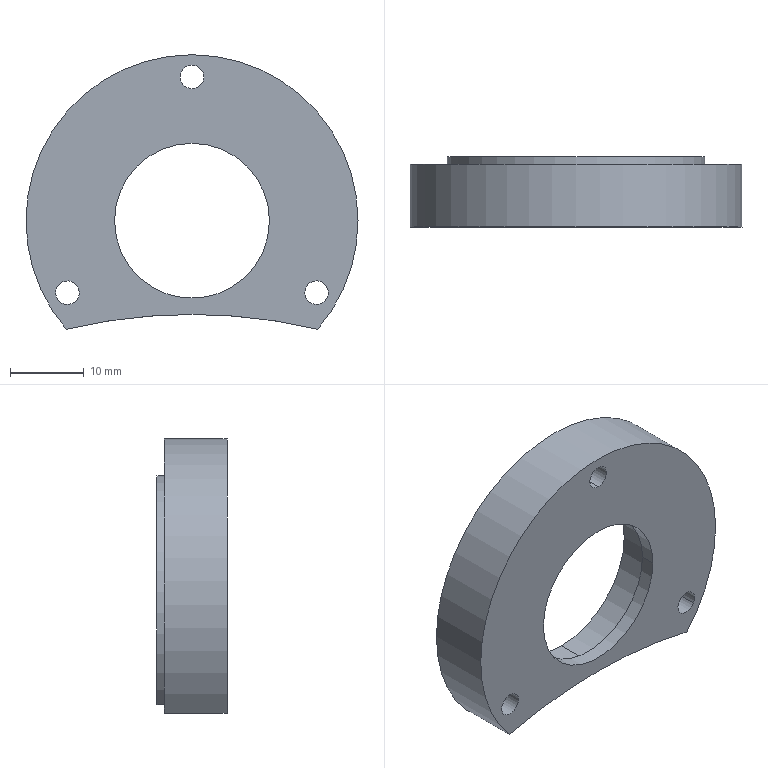CAM job | Mastercam | mm | 3 operations | part box 45 x 9.5 x 37.2
1. Contour (Ramp) | 13 - 16 平铣刀
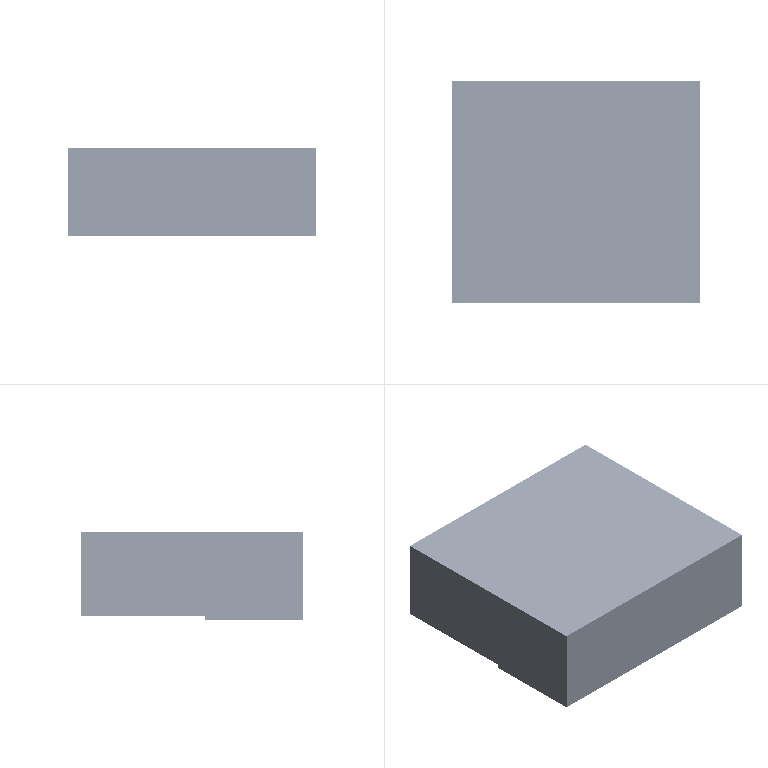2. Contour (2D) | 10 - 10 平铣刀
3. Drill/Counterbore | 5 - 4 倒角刀